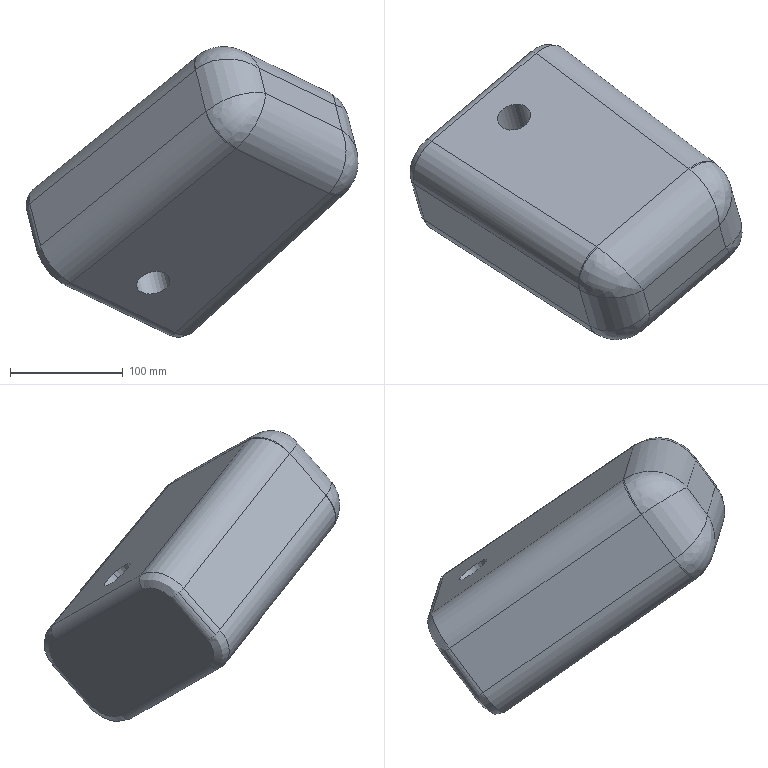Component | SolidWorks | Buffer Block^LandingGearAssembly-1 | 1 solid | 33 faces | volume 4719196 mm3 | cylinder 15 | spline 12 | plane 6 | commonest cylinder face diameters 20 x5 60 x4 80 x4 30 x2